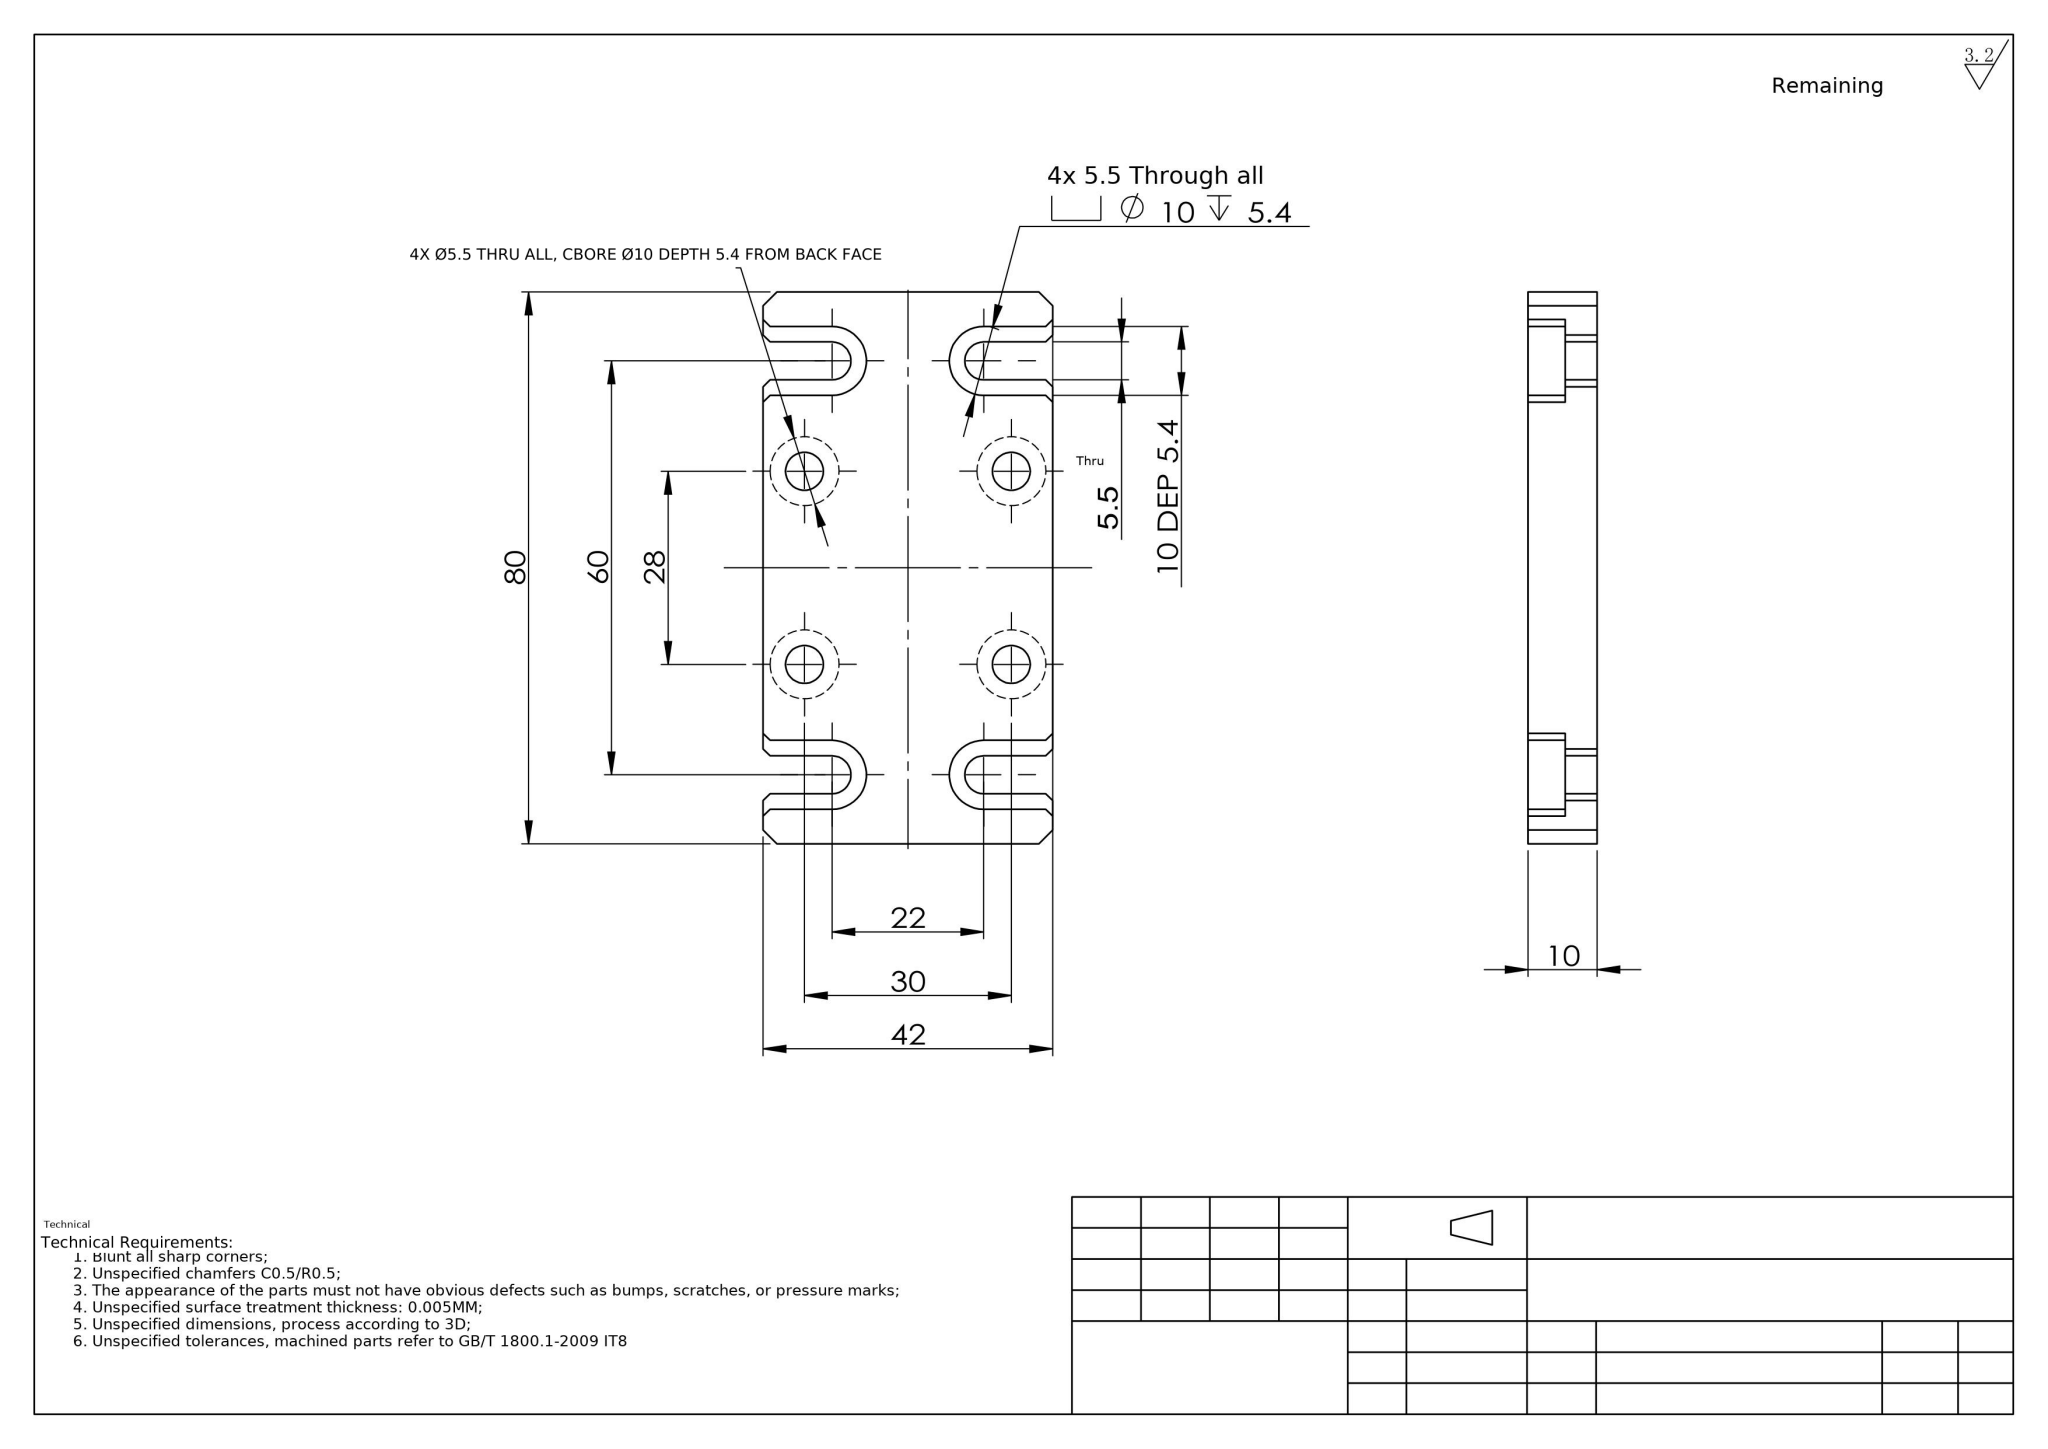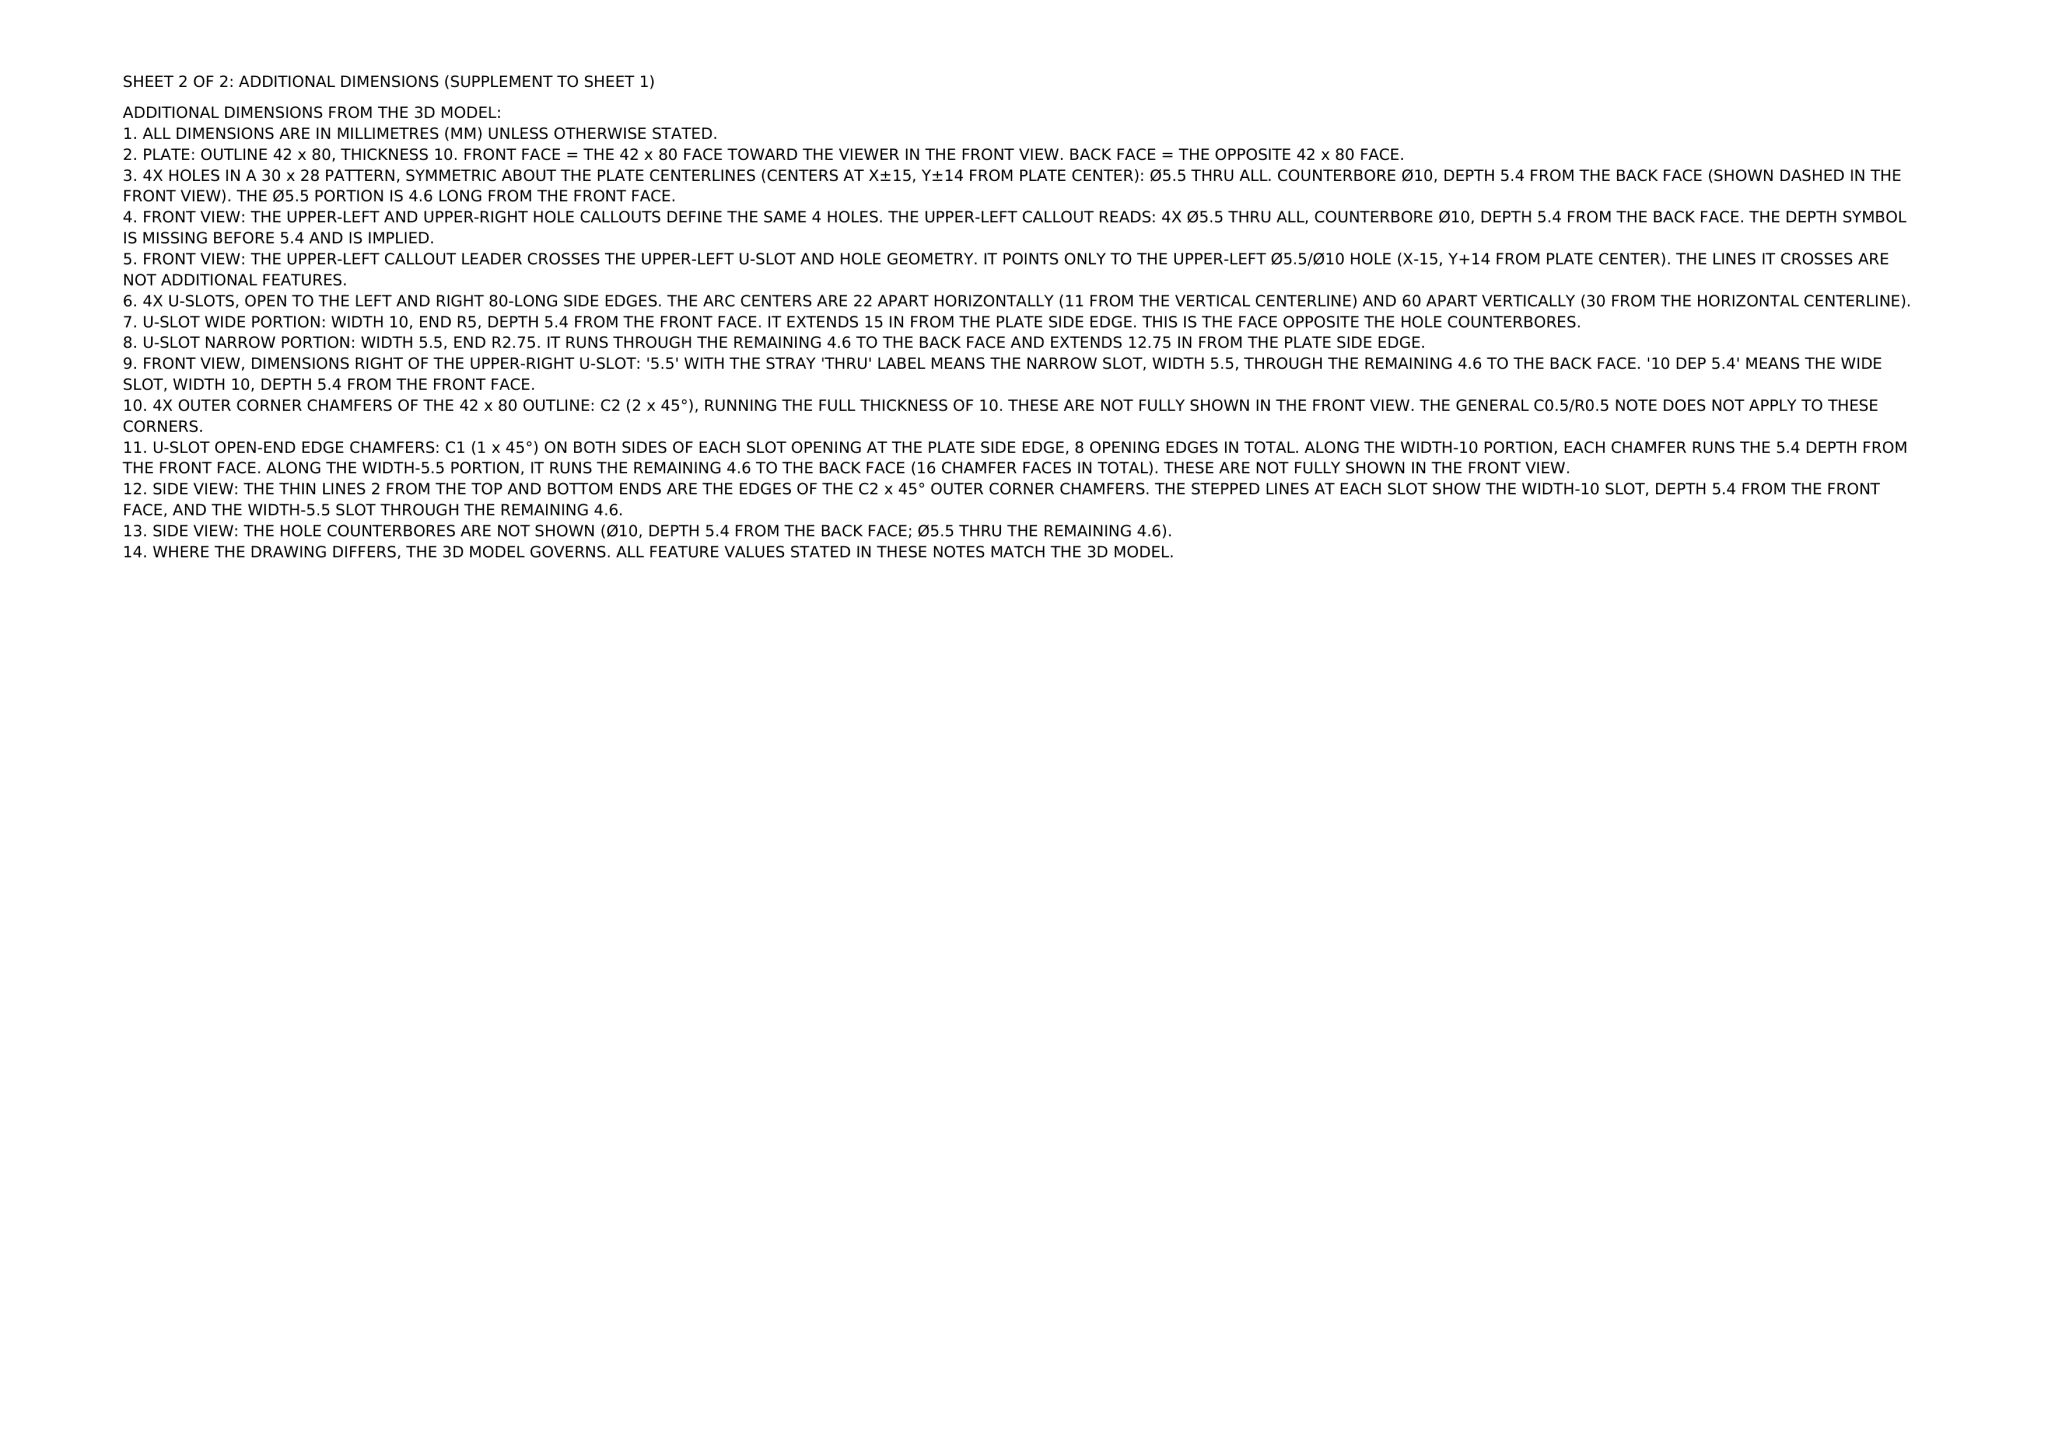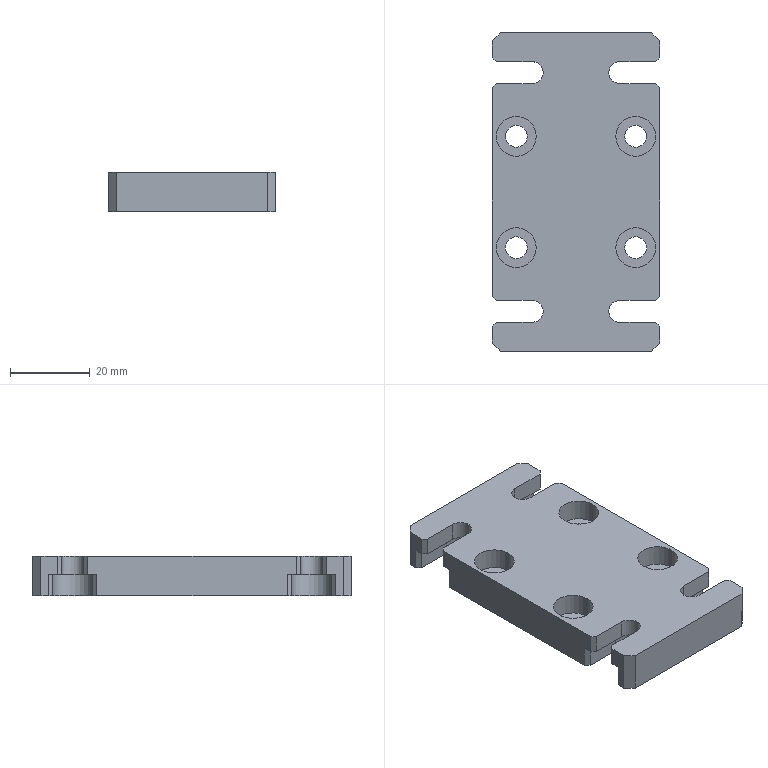Part | NX | mm | 1 solid | 82 faces | box 42 x 80 x 10 mm | volume 27108 mm3 | plane 54 | cylinder 28 | commonest cylinder face diameters 10 x14 5.5 x14